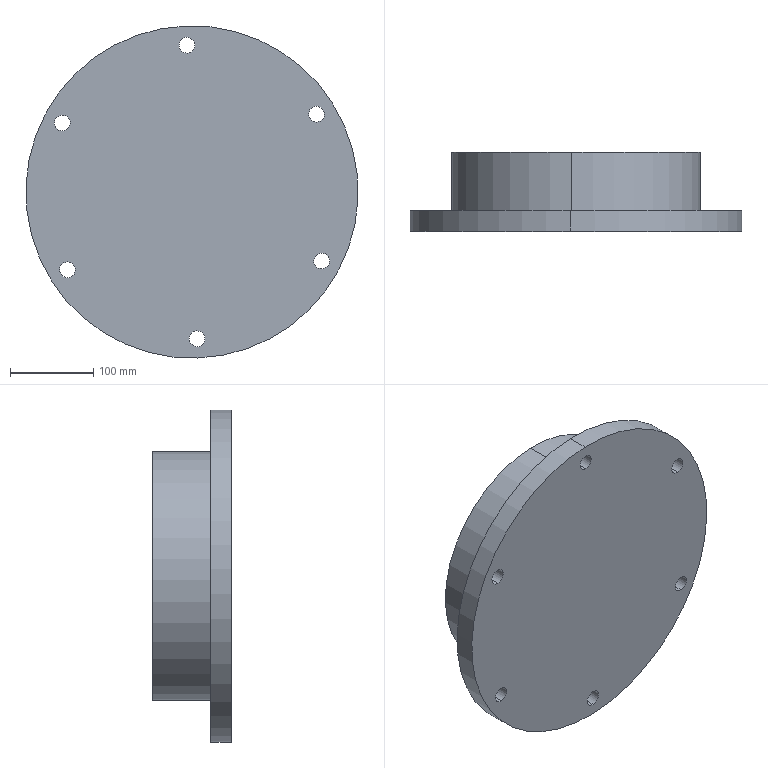Component | SolidWorks | Base-1 | 1 solid | 52 faces | box 400 x 95 x 400 mm | volume 7229203 mm3 | cylinder 32 | cone 12 | plane 8 | commonest cylinder face diameters 14 x12 19 x12 10 x4 400 x2 300 x2
build123d program:
from build123d import *

# Parameters (mm, degrees)
CIRPATTERN1_COUNT  = 6
SKETCH7_W          = 80
SKETCH7_H          = 165
CUT_EXTRUDE2_DEPTH = 60
CIRPATTERN2_COUNT  = 6
FILLET1_R          = 5


with BuildPart() as part:
    # Sketch1 → Revolve1 (revolve)
    with BuildSketch(Plane(origin=(0, 0, 0), x_dir=(0, 0, -1), z_dir=(1, 0, 0))):
        Polygon((0, 0), (150, 0), (150, -70), (200, -70), (200, -95), (0, -95), align=None)
    revolve(axis=Axis((0, -95, 0), (0, 1, 0)))

    # Sketch3 → 19.0 _19_ Diameter Hole1 (revolve, cut)
    with BuildSketch(Plane(origin=(0, -70, -176.862), x_dir=(0, 0, 1), z_dir=(1, 0, 0))):
        Polygon((0, 0), (0, 30.708), (9.5, 25), (9.5, 0), align=None)
    f_19_0_19_diameter_hole1 = revolve(axis=Axis((0, -63.65, -176.862), (0, -1, 0)), mode=Mode.SUBTRACT)

    # CirPattern1: 19.0 _19_ Diameter Hole1 ×6 about axis
    cirpattern1_axis = Axis((0, 0, 0), (0, 1, 0))
    for i in range(1, CIRPATTERN1_COUNT):
        add(f_19_0_19_diameter_hole1.rotate(cirpattern1_axis, i * 360 / CIRPATTERN1_COUNT), mode=Mode.SUBTRACT)

    # Sketch7 → Cut-Extrude2 (cut)
    with BuildSketch(Plane(origin=(0, 0, 0), x_dir=(1, 0, 0), z_dir=(0, 1, 0))):
        Rectangle(SKETCH7_W, SKETCH7_H)
    extrude(amount=-CUT_EXTRUDE2_DEPTH, mode=Mode.SUBTRACT)

    # Sketch10 → M14 Tapped Hole1 (revolve, cut)
    with BuildSketch(Plane(origin=(-120.833, 0, 32.282), x_dir=(0, 0, 1), z_dir=(1, 0, 0))):
        Polygon((0, 0), (0, 32.206), (7, 28), (7, 0), align=None)
    m14_tapped_hole1 = revolve(axis=Axis((-120.833, 6.35, 32.282), (0, -1, 0)), mode=Mode.SUBTRACT)

    # CirPattern2: M14 Tapped Hole1 ×6 about axis
    cirpattern2_axis = Axis((0, 0, 0), (0, 1, 0))
    for i in range(1, CIRPATTERN2_COUNT):
        add(m14_tapped_hole1.rotate(cirpattern2_axis, i * 360 / CIRPATTERN2_COUNT), mode=Mode.SUBTRACT)

    # Fillet1
    fillet1_edges = [part.edges().sort_by_distance(p)[0] for p in [
        (40, -30, -82.5),
        (40, -30, 82.5),
        (-40, -30, 82.5),
        (-40, -30, -82.5),
    ]]
    fillet(fillet1_edges, radius=FILLET1_R)


solid = part.part

# Placed as in the assembly
solid = solid.moved(Location((-87.309, 186.019, 566.392), (0, -2, 0)))